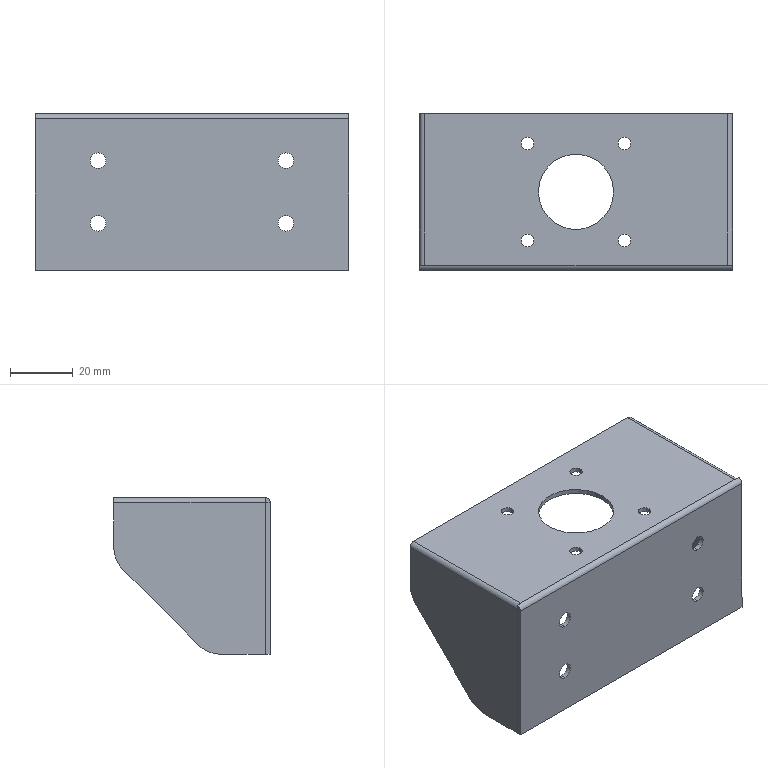Component | SolidWorks | MotorFixture-1 | 1 solid | 56 faces | volume 19475 mm3 | cylinder 28 | plane 28 | commonest cylinder face diameters 5 x8 4 x8 20 x4 3.2 x3 0.2 x3 24 x2